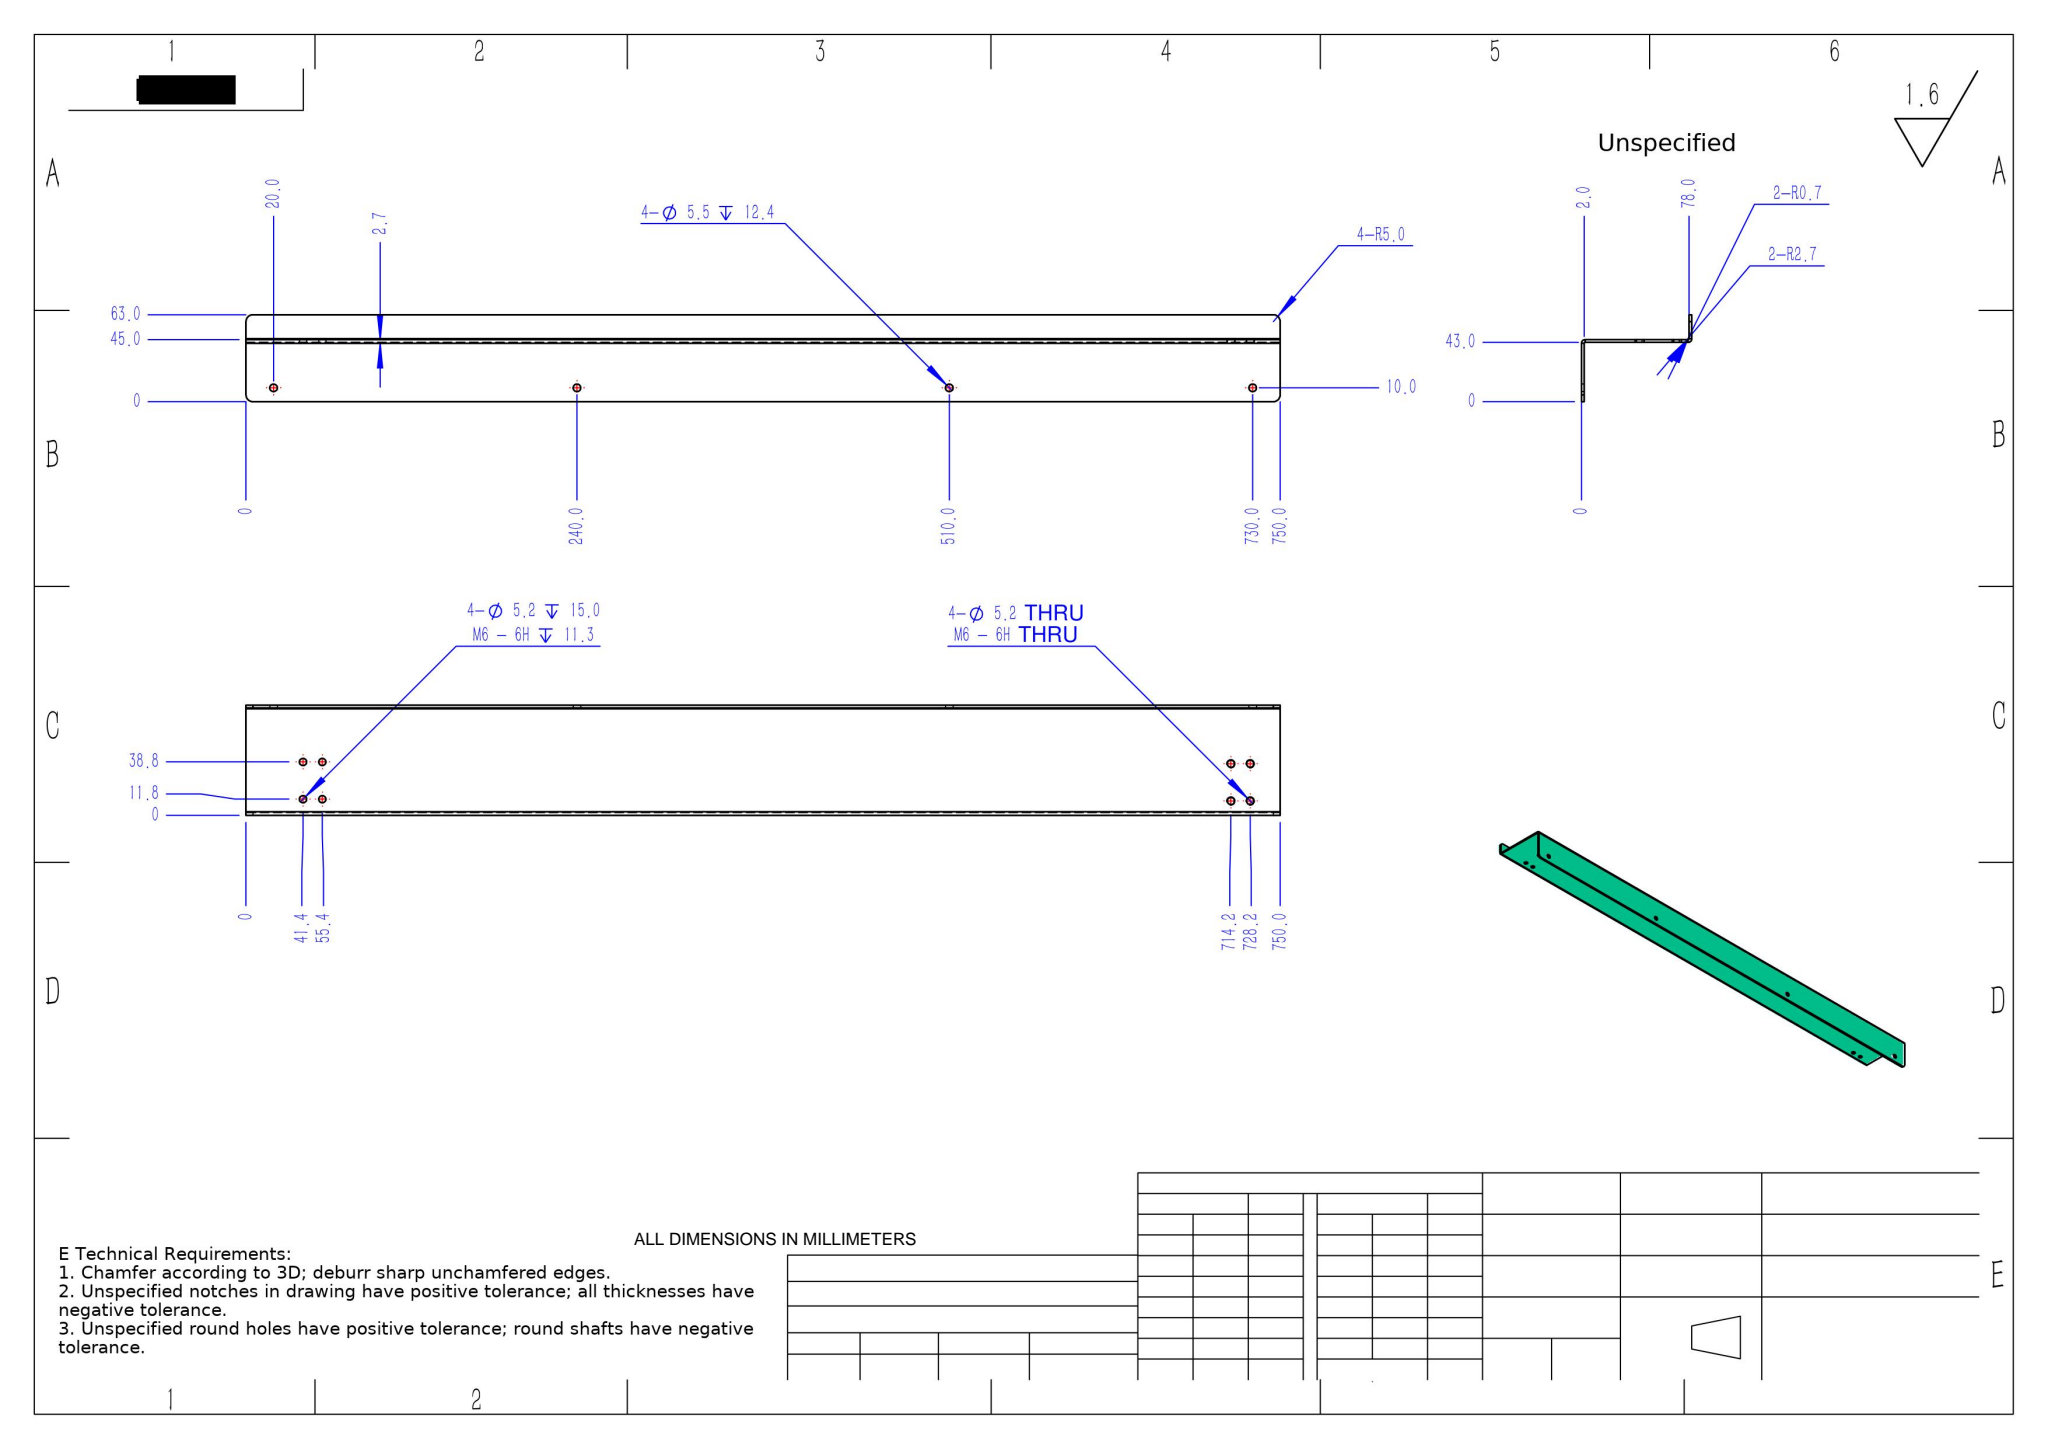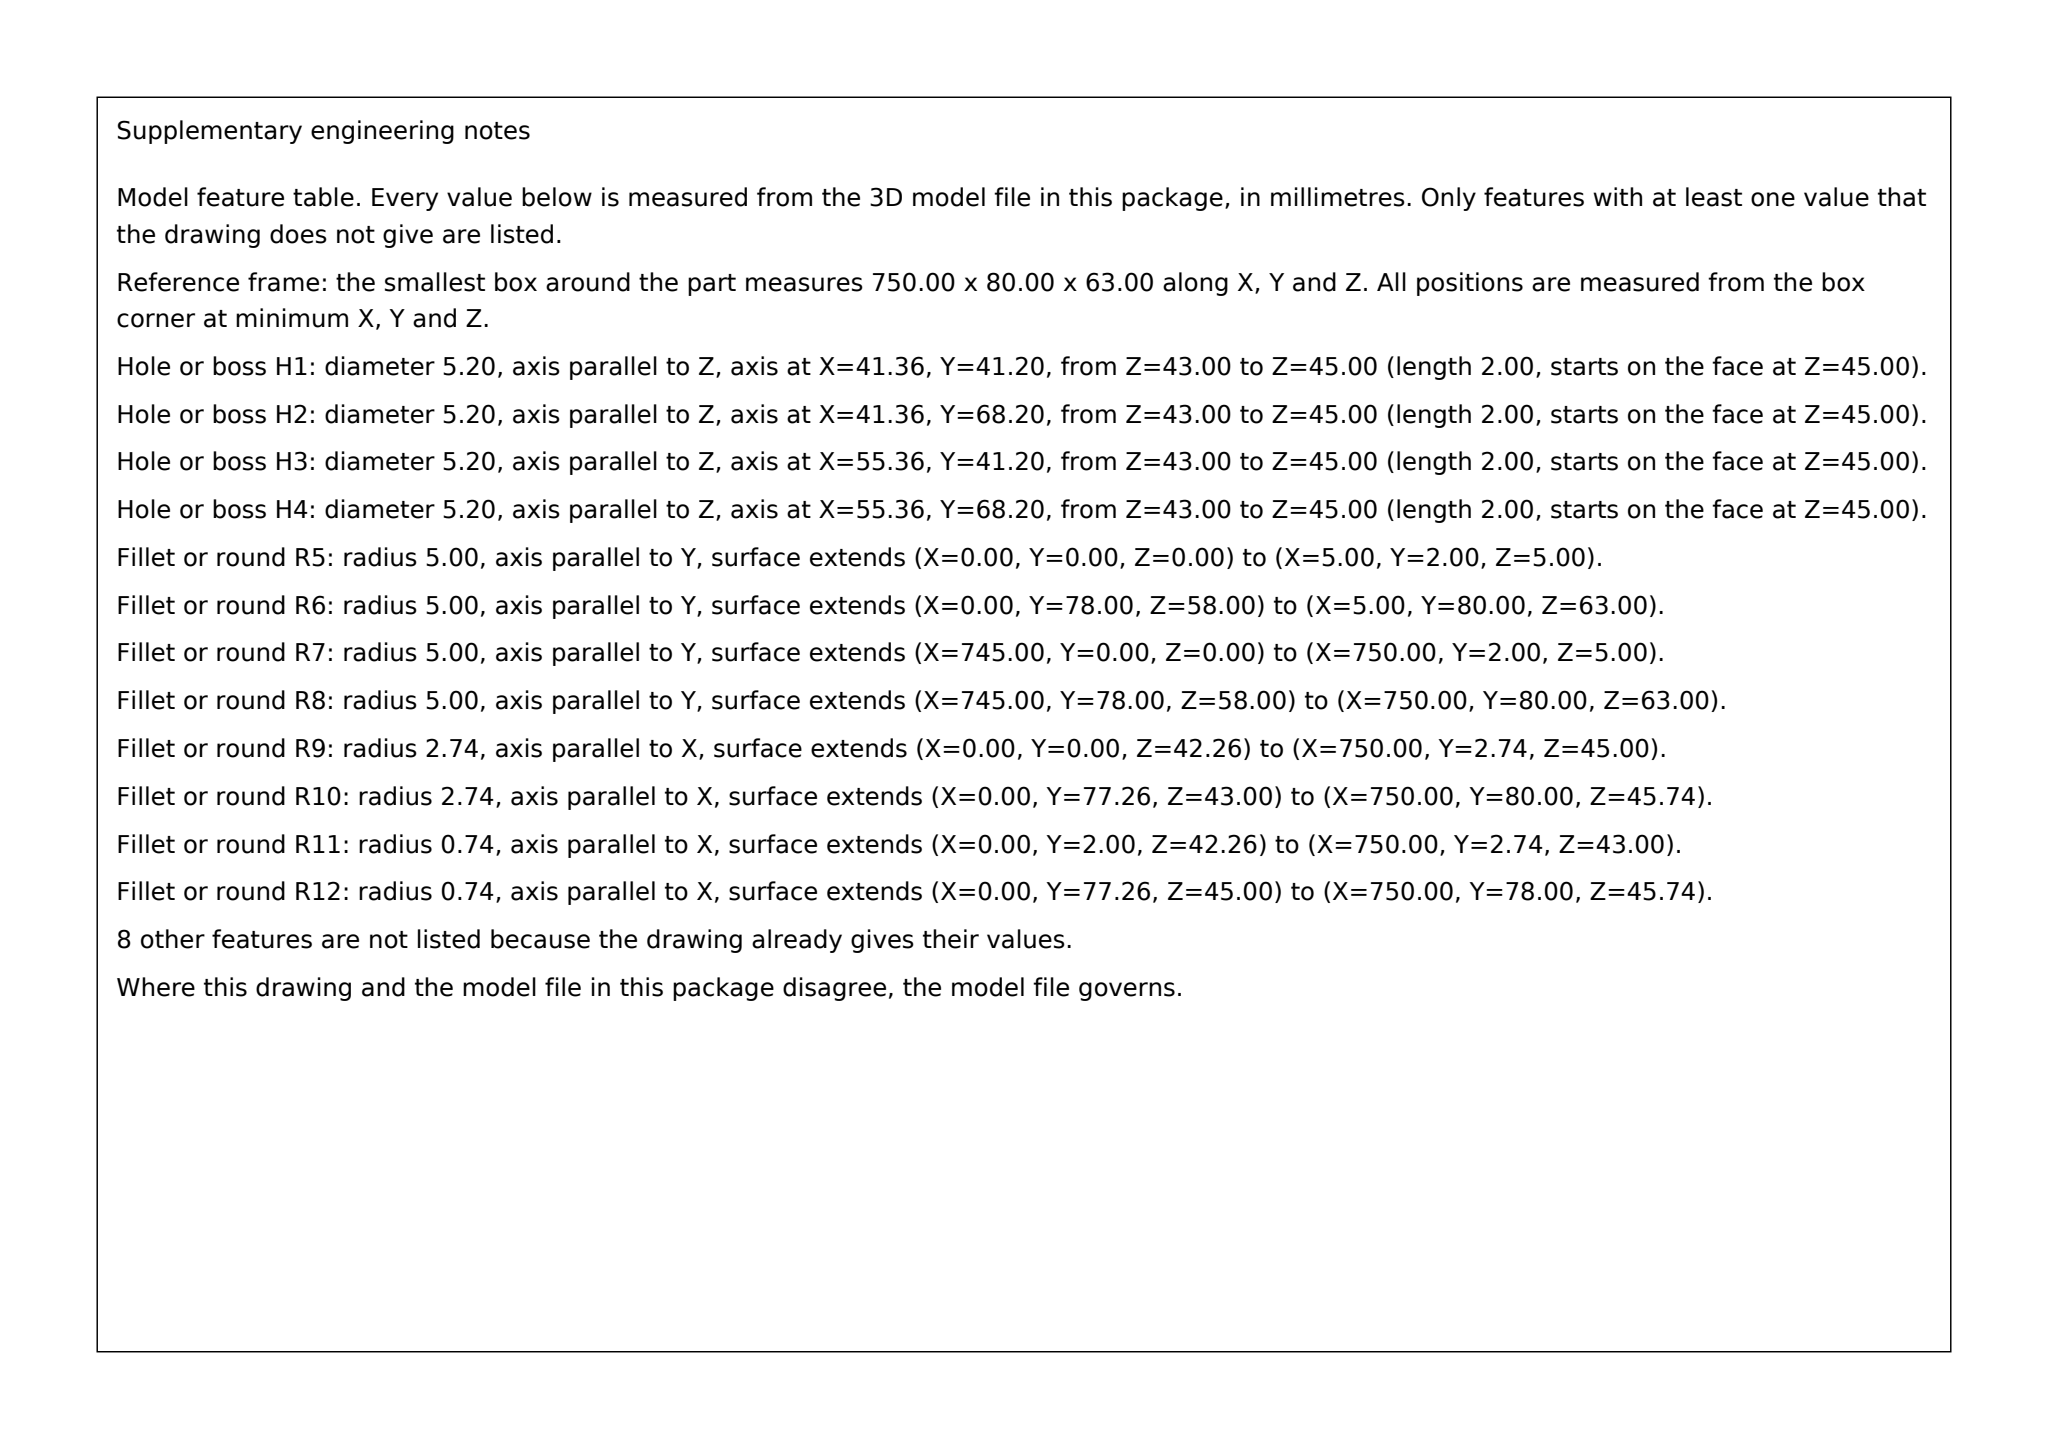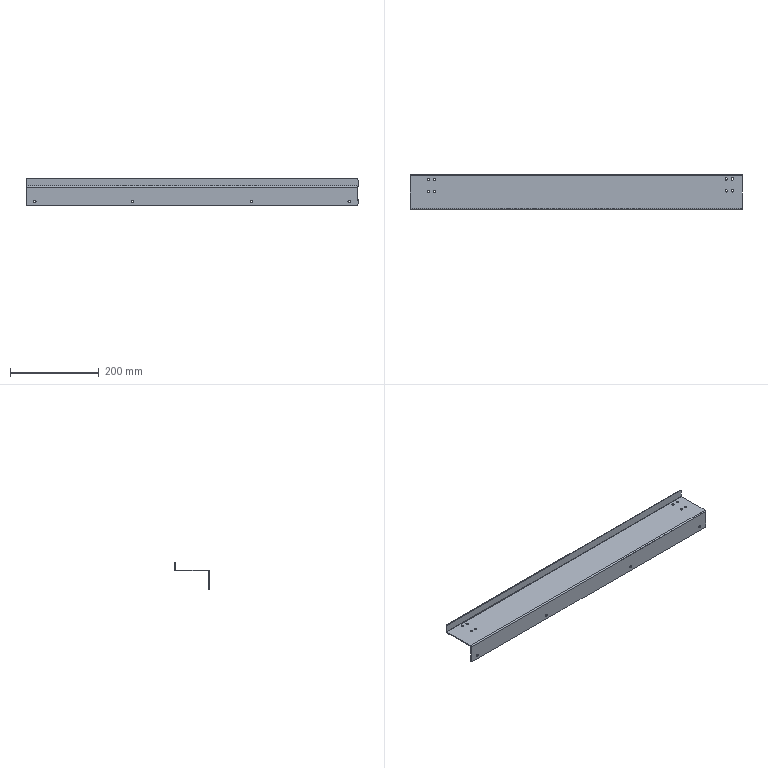Part | SolidWorks | mm | 1 solid | 50 faces | box 750 x 80 x 63 mm | volume 208691 mm3 | cylinder 32 | plane 18 | commonest cylinder face diameters 5.2 x16 5.5 x8 10 x4 5.473 x2 1.473 x2